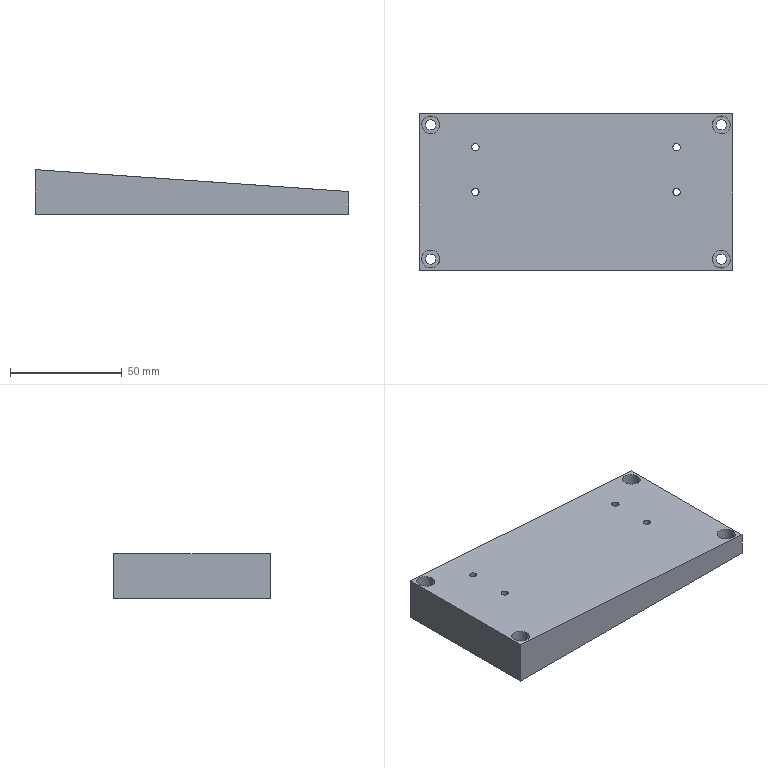Component | SolidWorks | CSFA2082 077-1 | 1 solid | 34 faces | box 140 x 70 x 20 mm | volume 145026 mm3 | cylinder 24 | plane 10 | commonest cylinder face diameters 3.3 x8 8 x8 4.5 x8
build123d program:
from build123d import *

# Parameters (mm, degrees)
SKETCH1_W          = 140
SKETCH1_H          = 70
EXTRUDE1_DEPTH     = 20
CUT_EXTRUDE1_DEPTH = 134
SKETCH3_R          = 2.25
CUT_EXTRUDE2_DEPTH = 68
CUT_EXTRUDE3_START = -4
SKETCH4_R          = 4
CUT_EXTRUDE3_DEPTH = 68
M4_TAPPED_HOLE1_D  = 3.3


with BuildPart() as part:
    # Sketch1 → Extrude1 (new body)
    with BuildSketch(Plane.XY):
        Rectangle(SKETCH1_W, SKETCH1_H)
    extrude(amount=EXTRUDE1_DEPTH)

    # Sketch2 → Cut-Extrude1 (cut)
    with BuildSketch(Plane.XZ.offset(35)):
        Polygon((-70, 20), (70, 10.21), (70, 20), align=None)
    extrude(amount=-CUT_EXTRUDE1_DEPTH, mode=Mode.SUBTRACT)

    # Sketch3 → Cut-Extrude2 (cut)
    with BuildSketch(Plane(origin=(0, 0, 0), x_dir=(-1, 0, 0), z_dir=(0, 0, -1))):
        with Locations((-65, 30)):
            Circle(SKETCH3_R)
        with Locations((65, 30)):
            Circle(SKETCH3_R)
        with Locations((-65, -30)):
            Circle(SKETCH3_R)
        with Locations((65, -30)):
            Circle(SKETCH3_R)
    extrude(amount=-CUT_EXTRUDE2_DEPTH, mode=Mode.SUBTRACT)

    # Sketch4 → Cut-Extrude3 (cut)
    with BuildSketch(Plane(origin=(0, 0, 0), x_dir=(-1, 0, 0), z_dir=(0, 0, -1)).offset(CUT_EXTRUDE3_START)):
        with Locations((-65, 30)):
            Circle(SKETCH4_R)
        with Locations((-65, -30)):
            Circle(SKETCH4_R)
        with Locations((65, -30)):
            Circle(SKETCH4_R)
        with Locations((65, 30)):
            Circle(SKETCH4_R)
    extrude(amount=-CUT_EXTRUDE3_DEPTH, mode=Mode.SUBTRACT)

    # M4 Tapped Hole1 (through all)
    with Locations(Plane(origin=(0, 0, 0), x_dir=(-1, 0, 0), z_dir=(0, 0, -1))):
        with Locations((-45, 20), (-45, 0), (45, 20), (45, 0)):
            Hole(M4_TAPPED_HOLE1_D / 2)


solid = part.part

# Placed as in the assembly
solid = solid.moved(Location((178.594, -218.176, 771), (0, 0, 0)))